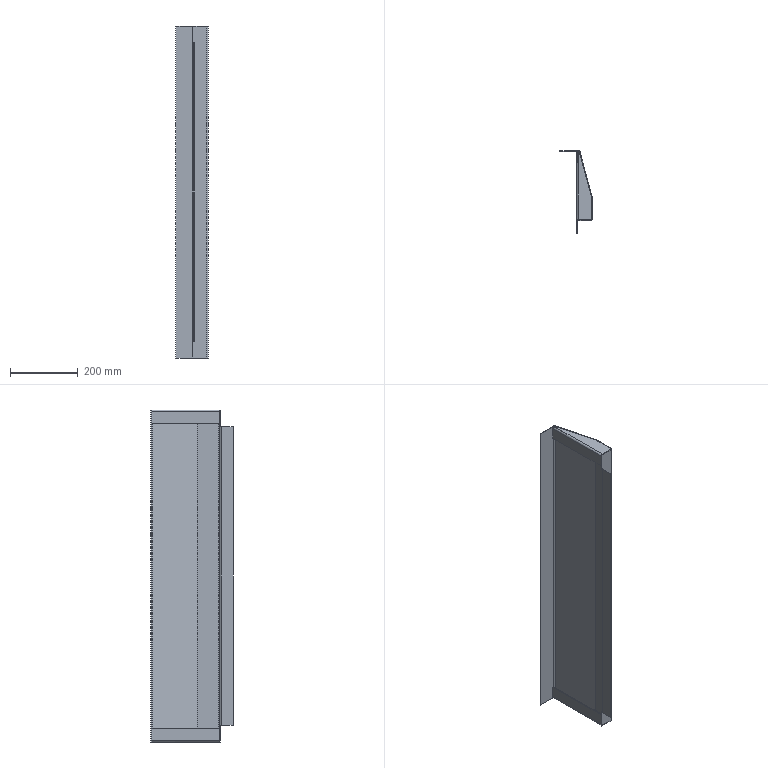Component | NX | UPPER_BEAM_REAR | 3 solids | 60 faces | volume 719027 mm3 | plane 44 | cylinder 16 | commonest cylinder face diameters 10 x8 6 x8